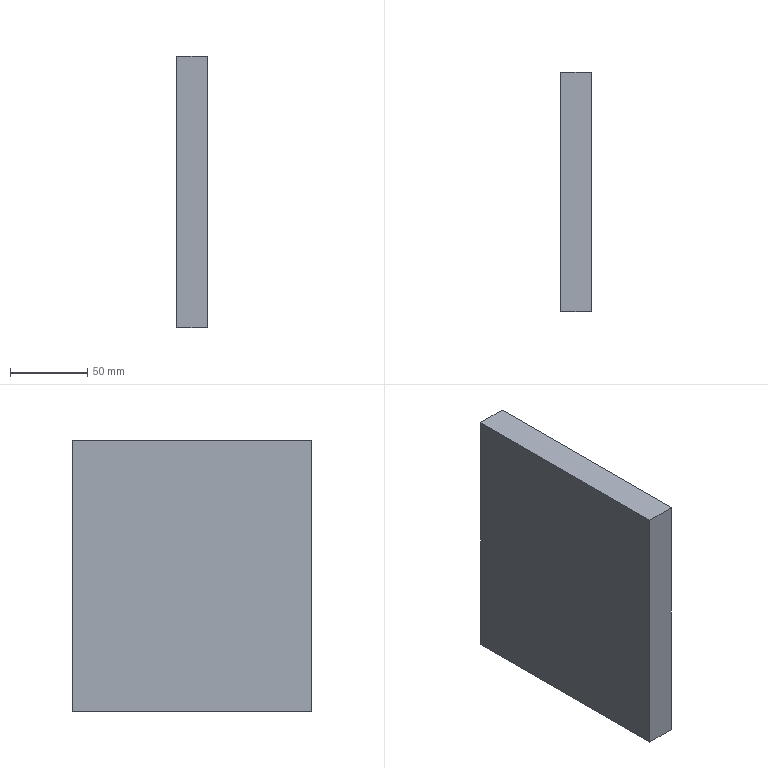Component | SolidWorks | MotorBasePlate-1 | 1 solid | 6 faces | box 20 x 155 x 176 mm | volume 545600 mm3 | plane 6 | material 45
build123d program:
from build123d import *

# Parameters (mm, degrees)
SKETCH1_W           = 176
SKETCH1_H           = 155
BOSS_EXTRUDE1_DEPTH = 20


with BuildPart() as part:
    # Sketch1 → Boss-Extrude1 (new body)
    with BuildSketch(Plane(origin=(0, 0, 0), x_dir=(1, 0, 0), z_dir=(0, 1, 0))):
        Rectangle(SKETCH1_W, SKETCH1_H)
    extrude(amount=BOSS_EXTRUDE1_DEPTH)


solid = part.part

# Placed as in the assembly
solid = solid.moved(Location((-261.359, -208.685, 1412), (90, 0, 90)))
STEP:
#1=COLOUR_RGB('',0.7922,0.8196,0.9333);
#2=FILL_AREA_STYLE_COLOUR('',#1);
#3=FILL_AREA_STYLE('',(#2));
#4=SURFACE_STYLE_FILL_AREA(#3);
#5=SURFACE_SIDE_STYLE('',(#4));
#6=SURFACE_STYLE_USAGE(.BOTH.,#5);
#7=PRESENTATION_STYLE_ASSIGNMENT((#6));
#8=CARTESIAN_POINT('',(-10.29,-5.165,52.126));
#9=VERTEX_POINT('',#8);
#10=CARTESIAN_POINT('',(-10.29,-11.267,52.126));
#11=VERTEX_POINT('',#10);
#12=CARTESIAN_POINT('',(-10.29,-11.267,52.126));
#13=DIRECTION('',(0.,-1.,0.));
#14=VECTOR('',#13,39.37);
#15=LINE('',#12,#14);
#16=EDGE_CURVE('',#9,#11,#15,.T.);
#17=ORIENTED_EDGE('',*,*,#16,.T.);
#18=CARTESIAN_POINT('',(-11.077,-11.267,52.126));
#19=VERTEX_POINT('',#18);
#20=CARTESIAN_POINT('',(-11.077,-11.267,52.126));
#21=DIRECTION('',(1.,-0.,0.));
#22=VECTOR('',#21,39.37);
#23=LINE('',#20,#22);
#24=EDGE_CURVE('',#19,#11,#23,.T.);
#25=ORIENTED_EDGE('',*,*,#24,.F.);
#26=CARTESIAN_POINT('',(-11.077,-5.165,52.126));
#27=VERTEX_POINT('',#26);
#28=CARTESIAN_POINT('',(-11.077,-11.267,52.126));
#29=DIRECTION('',(0.,-1.,0.));
#30=VECTOR('',#29,39.37);
#31=LINE('',#28,#30);
#32=EDGE_CURVE('',#27,#19,#31,.T.);
#33=ORIENTED_EDGE('',*,*,#32,.F.);
#34=CARTESIAN_POINT('',(-11.077,-5.165,52.126));
#35=DIRECTION('',(1.,-0.,0.));
#36=VECTOR('',#35,39.37);
#37=LINE('',#34,#36);
#38=EDGE_CURVE('',#27,#9,#37,.T.);
#39=ORIENTED_EDGE('',*,*,#38,.T.);
#40=EDGE_LOOP('',(#17,#25,#33,#39));
#41=FACE_OUTER_BOUND('',#40,.T.);
#42=CARTESIAN_POINT('',(-11.077,-11.267,52.126));
#43=DIRECTION('',(-0.,0.,1.));
#44=DIRECTION('',(-0.,1.,-0.));
#45=AXIS2_PLACEMENT_3D('',#42,#43,#44);
#46=PLANE('',#45);
#47=ADVANCED_FACE('',(#41),#46,.F.);
#48=CARTESIAN_POINT('',(-10.29,-11.267,59.055));
#49=VERTEX_POINT('',#48);
#50=CARTESIAN_POINT('',(-10.29,-11.267,59.055));
#51=DIRECTION('',(-0.,0.,1.));
#52=VECTOR('',#51,39.37);
#53=LINE('',#50,#52);
#54=EDGE_CURVE('',#11,#49,#53,.T.);
#55=ORIENTED_EDGE('',*,*,#54,.T.);
#56=CARTESIAN_POINT('',(-11.077,-11.267,59.055));
#57=VERTEX_POINT('',#56);
#58=CARTESIAN_POINT('',(-11.077,-11.267,59.055));
#59=DIRECTION('',(1.,-0.,0.));
#60=VECTOR('',#59,39.37);
#61=LINE('',#58,#60);
#62=EDGE_CURVE('',#57,#49,#61,.T.);
#63=ORIENTED_EDGE('',*,*,#62,.F.);
#64=CARTESIAN_POINT('',(-11.077,-11.267,59.055));
#65=DIRECTION('',(-0.,0.,1.));
#66=VECTOR('',#65,39.37);
#67=LINE('',#64,#66);
#68=EDGE_CURVE('',#19,#57,#67,.T.);
#69=ORIENTED_EDGE('',*,*,#68,.F.);
#70=ORIENTED_EDGE('',*,*,#24,.T.);
#71=EDGE_LOOP('',(#55,#63,#69,#70));
#72=FACE_OUTER_BOUND('',#71,.T.);
#73=CARTESIAN_POINT('',(-11.077,-11.267,59.055));
#74=DIRECTION('',(-0.,1.,-0.));
#75=DIRECTION('',(0.,-0.,-1.));
#76=AXIS2_PLACEMENT_3D('',#73,#74,#75);
#77=PLANE('',#76);
#78=ADVANCED_FACE('',(#72),#77,.F.);
#79=CARTESIAN_POINT('',(-10.29,-5.165,59.055));
#80=VERTEX_POINT('',#79);
#81=CARTESIAN_POINT('',(-10.29,-11.267,59.055));
#82=DIRECTION('',(-0.,1.,-0.));
#83=VECTOR('',#82,39.37);
#84=LINE('',#81,#83);
#85=EDGE_CURVE('',#49,#80,#84,.T.);
#86=ORIENTED_EDGE('',*,*,#85,.T.);
#87=CARTESIAN_POINT('',(-11.077,-5.165,59.055));
#88=VERTEX_POINT('',#87);
#89=CARTESIAN_POINT('',(-11.077,-5.165,59.055));
#90=DIRECTION('',(1.,-0.,0.));
#91=VECTOR('',#90,39.37);
#92=LINE('',#89,#91);
#93=EDGE_CURVE('',#88,#80,#92,.T.);
#94=ORIENTED_EDGE('',*,*,#93,.F.);
#95=CARTESIAN_POINT('',(-11.077,-11.267,59.055));
#96=DIRECTION('',(-0.,1.,-0.));
#97=VECTOR('',#96,39.37);
#98=LINE('',#95,#97);
#99=EDGE_CURVE('',#57,#88,#98,.T.);
#100=ORIENTED_EDGE('',*,*,#99,.F.);
#101=ORIENTED_EDGE('',*,*,#62,.T.);
#102=EDGE_LOOP('',(#86,#94,#100,#101));
#103=FACE_OUTER_BOUND('',#102,.T.);
#104=CARTESIAN_POINT('',(-11.077,-11.267,59.055));
#105=DIRECTION('',(0.,-0.,-1.));
#106=DIRECTION('',(0.,-1.,0.));
#107=AXIS2_PLACEMENT_3D('',#104,#105,#106);
#108=PLANE('',#107);
#109=ADVANCED_FACE('',(#103),#108,.F.);
#110=CARTESIAN_POINT('',(-10.29,-5.165,59.055));
#111=DIRECTION('',(0.,0.,-1.));
#112=VECTOR('',#111,39.37);
#113=LINE('',#110,#112);
#114=EDGE_CURVE('',#80,#9,#113,.T.);
#115=ORIENTED_EDGE('',*,*,#114,.T.);
#116=ORIENTED_EDGE('',*,*,#38,.F.);
#117=CARTESIAN_POINT('',(-11.077,-5.165,59.055));
#118=DIRECTION('',(0.,0.,-1.));
#119=VECTOR('',#118,39.37);
#120=LINE('',#117,#119);
#121=EDGE_CURVE('',#88,#27,#120,.T.);
#122=ORIENTED_EDGE('',*,*,#121,.F.);
#123=ORIENTED_EDGE('',*,*,#93,.T.);
#124=EDGE_LOOP('',(#115,#116,#122,#123));
#125=FACE_OUTER_BOUND('',#124,.T.);
#126=CARTESIAN_POINT('',(-11.077,-5.165,59.055));
#127=DIRECTION('',(0.,-1.,-0.));
#128=DIRECTION('',(-0.,-0.,1.));
#129=AXIS2_PLACEMENT_3D('',#126,#127,#128);
#130=PLANE('',#129);
#131=ADVANCED_FACE('',(#125),#130,.F.);
#132=ORIENTED_EDGE('',*,*,#32,.T.);
#133=ORIENTED_EDGE('',*,*,#68,.T.);
#134=ORIENTED_EDGE('',*,*,#99,.T.);
#135=ORIENTED_EDGE('',*,*,#121,.T.);
#136=EDGE_LOOP('',(#132,#133,#134,#135));
#137=FACE_OUTER_BOUND('',#136,.T.);
#138=CARTESIAN_POINT('',(-11.077,-8.216,55.591));
#139=DIRECTION('',(-1.,0.,-0.));
#140=DIRECTION('',(0.,-1.,-0.));
#141=AXIS2_PLACEMENT_3D('',#138,#139,#140);
#142=PLANE('',#141);
#143=ADVANCED_FACE('',(#137),#142,.T.);
#144=ORIENTED_EDGE('',*,*,#16,.F.);
#145=ORIENTED_EDGE('',*,*,#114,.F.);
#146=ORIENTED_EDGE('',*,*,#85,.F.);
#147=ORIENTED_EDGE('',*,*,#54,.F.);
#148=EDGE_LOOP('',(#144,#145,#146,#147));
#149=FACE_OUTER_BOUND('',#148,.T.);
#150=CARTESIAN_POINT('',(-10.29,-8.216,55.591));
#151=DIRECTION('',(-1.,0.,-0.));
#152=DIRECTION('',(0.,-1.,-0.));
#153=AXIS2_PLACEMENT_3D('',#150,#151,#152);
#154=PLANE('',#153);
#155=ADVANCED_FACE('',(#149),#154,.F.);
#156=CLOSED_SHELL('',(#47,#78,#109,#131,#143,#155));
#157=MANIFOLD_SOLID_BREP('',#156);
#158=STYLED_ITEM('',(#7),#157);
#159=(LENGTH_UNIT()NAMED_UNIT(*)SI_UNIT($,.METRE.));
#160=LENGTH_MEASURE_WITH_UNIT(LENGTH_MEASURE(0.0254),#159);
#161=DIMENSIONAL_EXPONENTS(1.,0.,0.,0.,0.,0.,0.);
#162=(CONVERSION_BASED_UNIT('',#160)LENGTH_UNIT()NAMED_UNIT(#161));
#163=UNCERTAINTY_MEASURE_WITH_UNIT(LENGTH_MEASURE(0.00001),#162,'','');
#164=(NAMED_UNIT(*)PLANE_ANGLE_UNIT()SI_UNIT($,.RADIAN.));
#165=(NAMED_UNIT(*)SI_UNIT($,.STERADIAN.)SOLID_ANGLE_UNIT());
#166=(GEOMETRIC_REPRESENTATION_CONTEXT(3)GLOBAL_UNCERTAINTY_ASSIGNED_CONTEXT((#163))GLOBAL_UNIT_ASSIGNED_CONTEXT((#162,#164,#165))REPRESENTATION_CONTEXT('',''));
#167=MECHANICAL_DESIGN_GEOMETRIC_PRESENTATION_REPRESENTATION('',(#158),#166);
#168=PRESENTATION_LAYER_ASSIGNMENT('','',(#158));
#169=CARTESIAN_POINT('',(0.,0.,0.));
#170=DIRECTION('',(0.,0.,1.));
#171=DIRECTION('',(1.,0.,0.));
#172=AXIS2_PLACEMENT_3D('',#169,#170,#171);
#173=(LENGTH_UNIT()NAMED_UNIT(*)SI_UNIT($,.METRE.));
#174=LENGTH_MEASURE_WITH_UNIT(LENGTH_MEASURE(0.0254),#173);
#175=DIMENSIONAL_EXPONENTS(1.,0.,0.,0.,0.,0.,0.);
#176=(CONVERSION_BASED_UNIT('',#174)LENGTH_UNIT()NAMED_UNIT(#175));
#177=UNCERTAINTY_MEASURE_WITH_UNIT(LENGTH_MEASURE(0.00001),#176,'','');
#178=(NAMED_UNIT(*)PLANE_ANGLE_UNIT()SI_UNIT($,.RADIAN.));
#179=(NAMED_UNIT(*)SI_UNIT($,.STERADIAN.)SOLID_ANGLE_UNIT());
#180=(GEOMETRIC_REPRESENTATION_CONTEXT(3)GLOBAL_UNCERTAINTY_ASSIGNED_CONTEXT((#177))GLOBAL_UNIT_ASSIGNED_CONTEXT((#176,#178,#179))REPRESENTATION_CONTEXT('',''));
#181=ADVANCED_BREP_SHAPE_REPRESENTATION('',(#157,#172),#180);